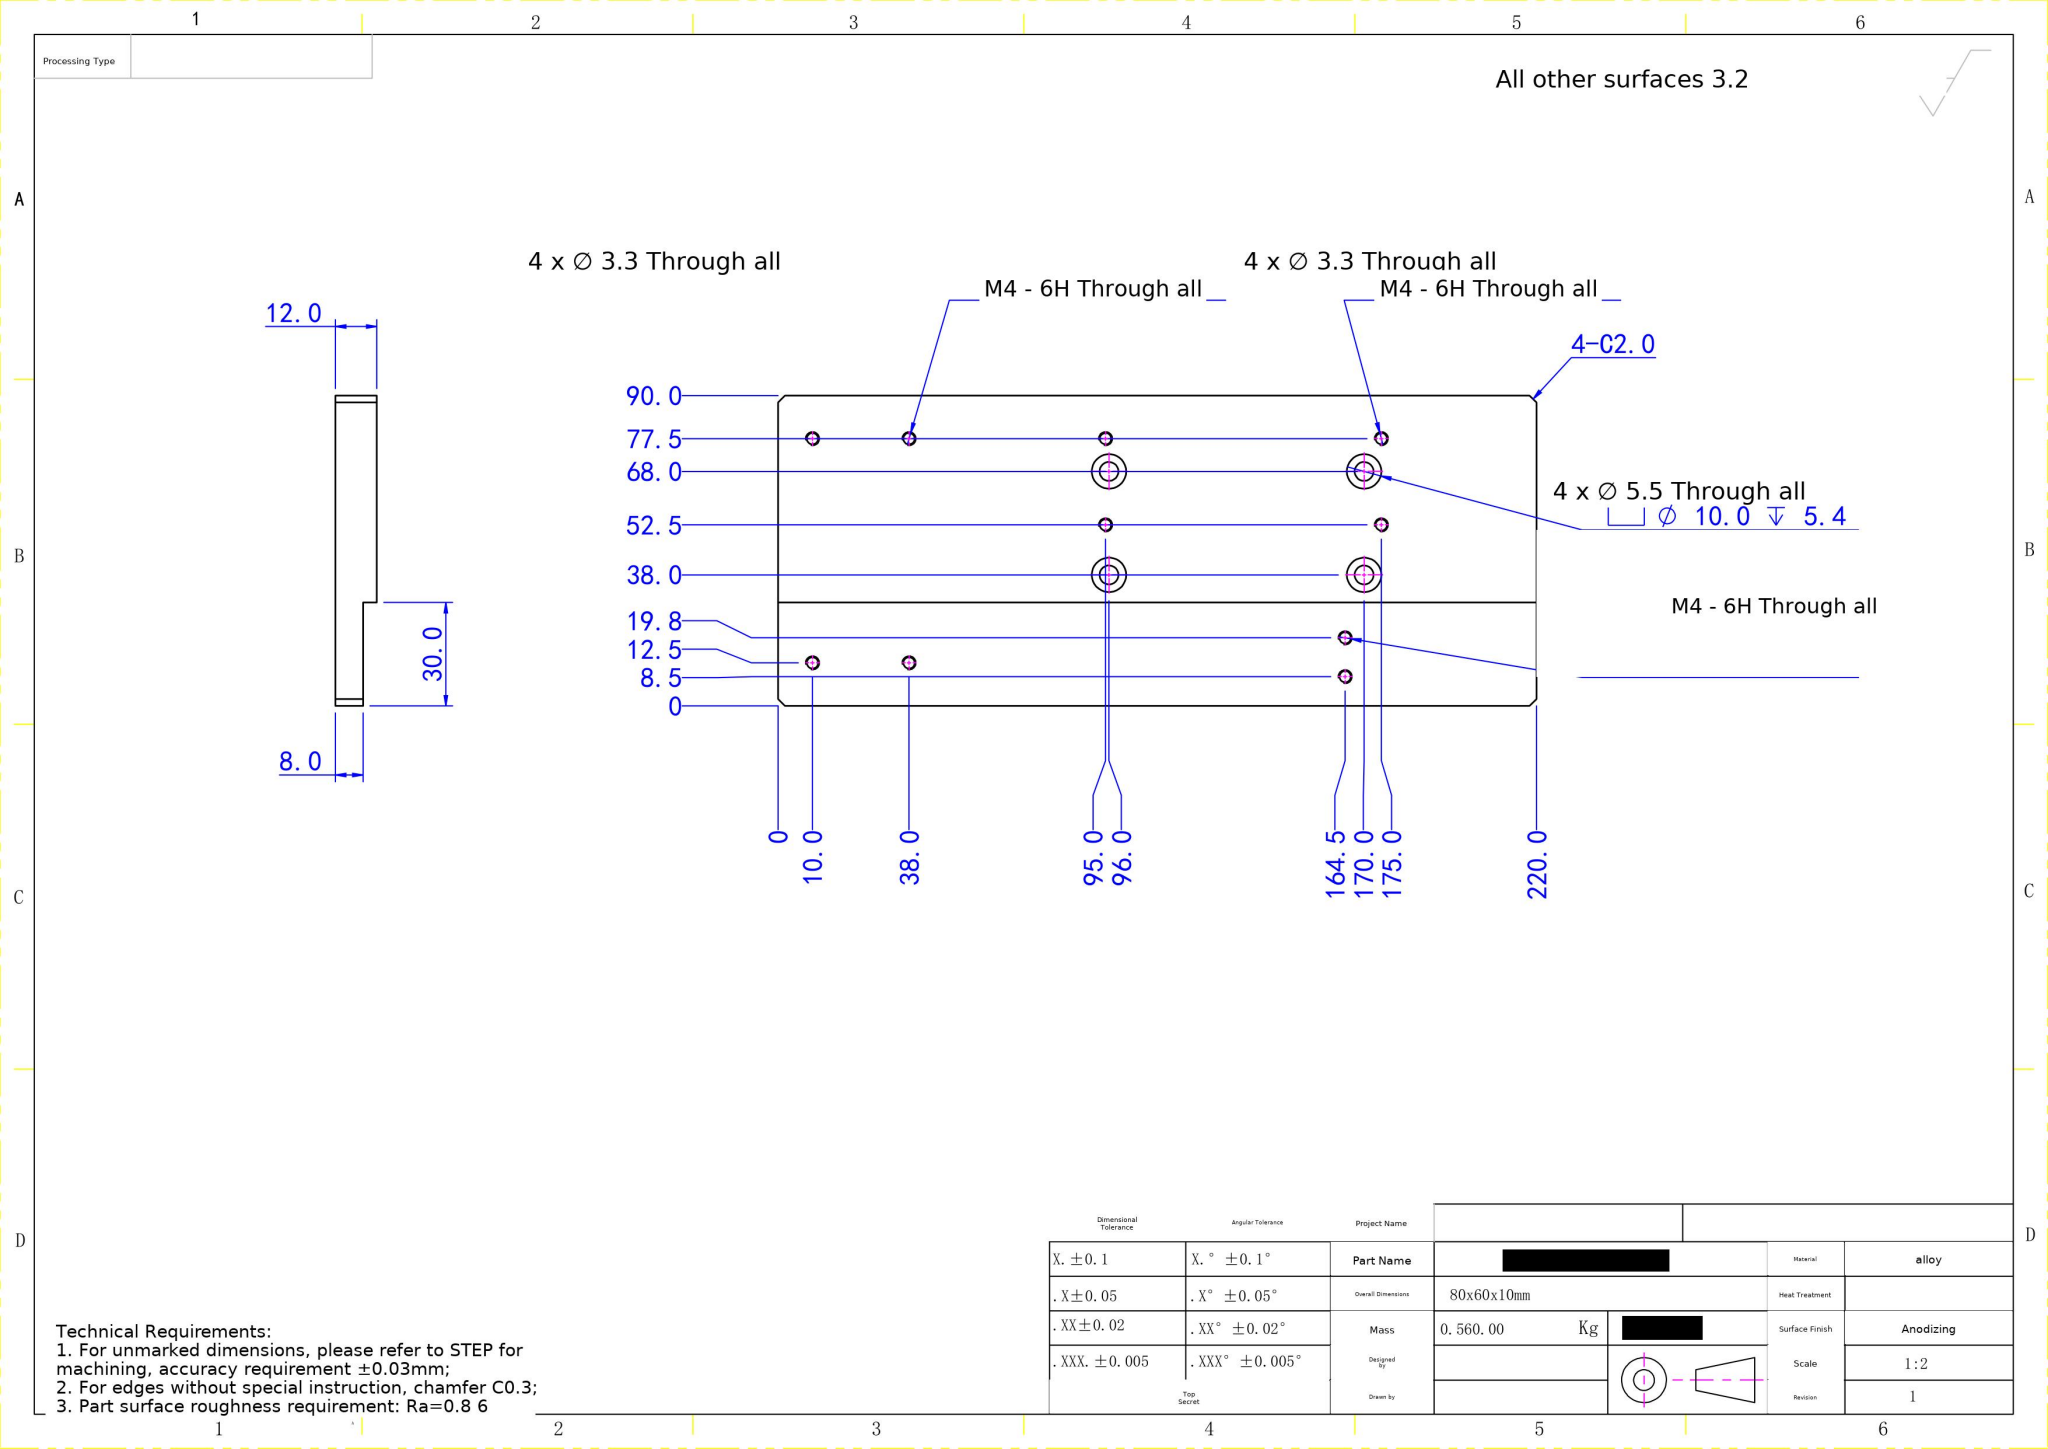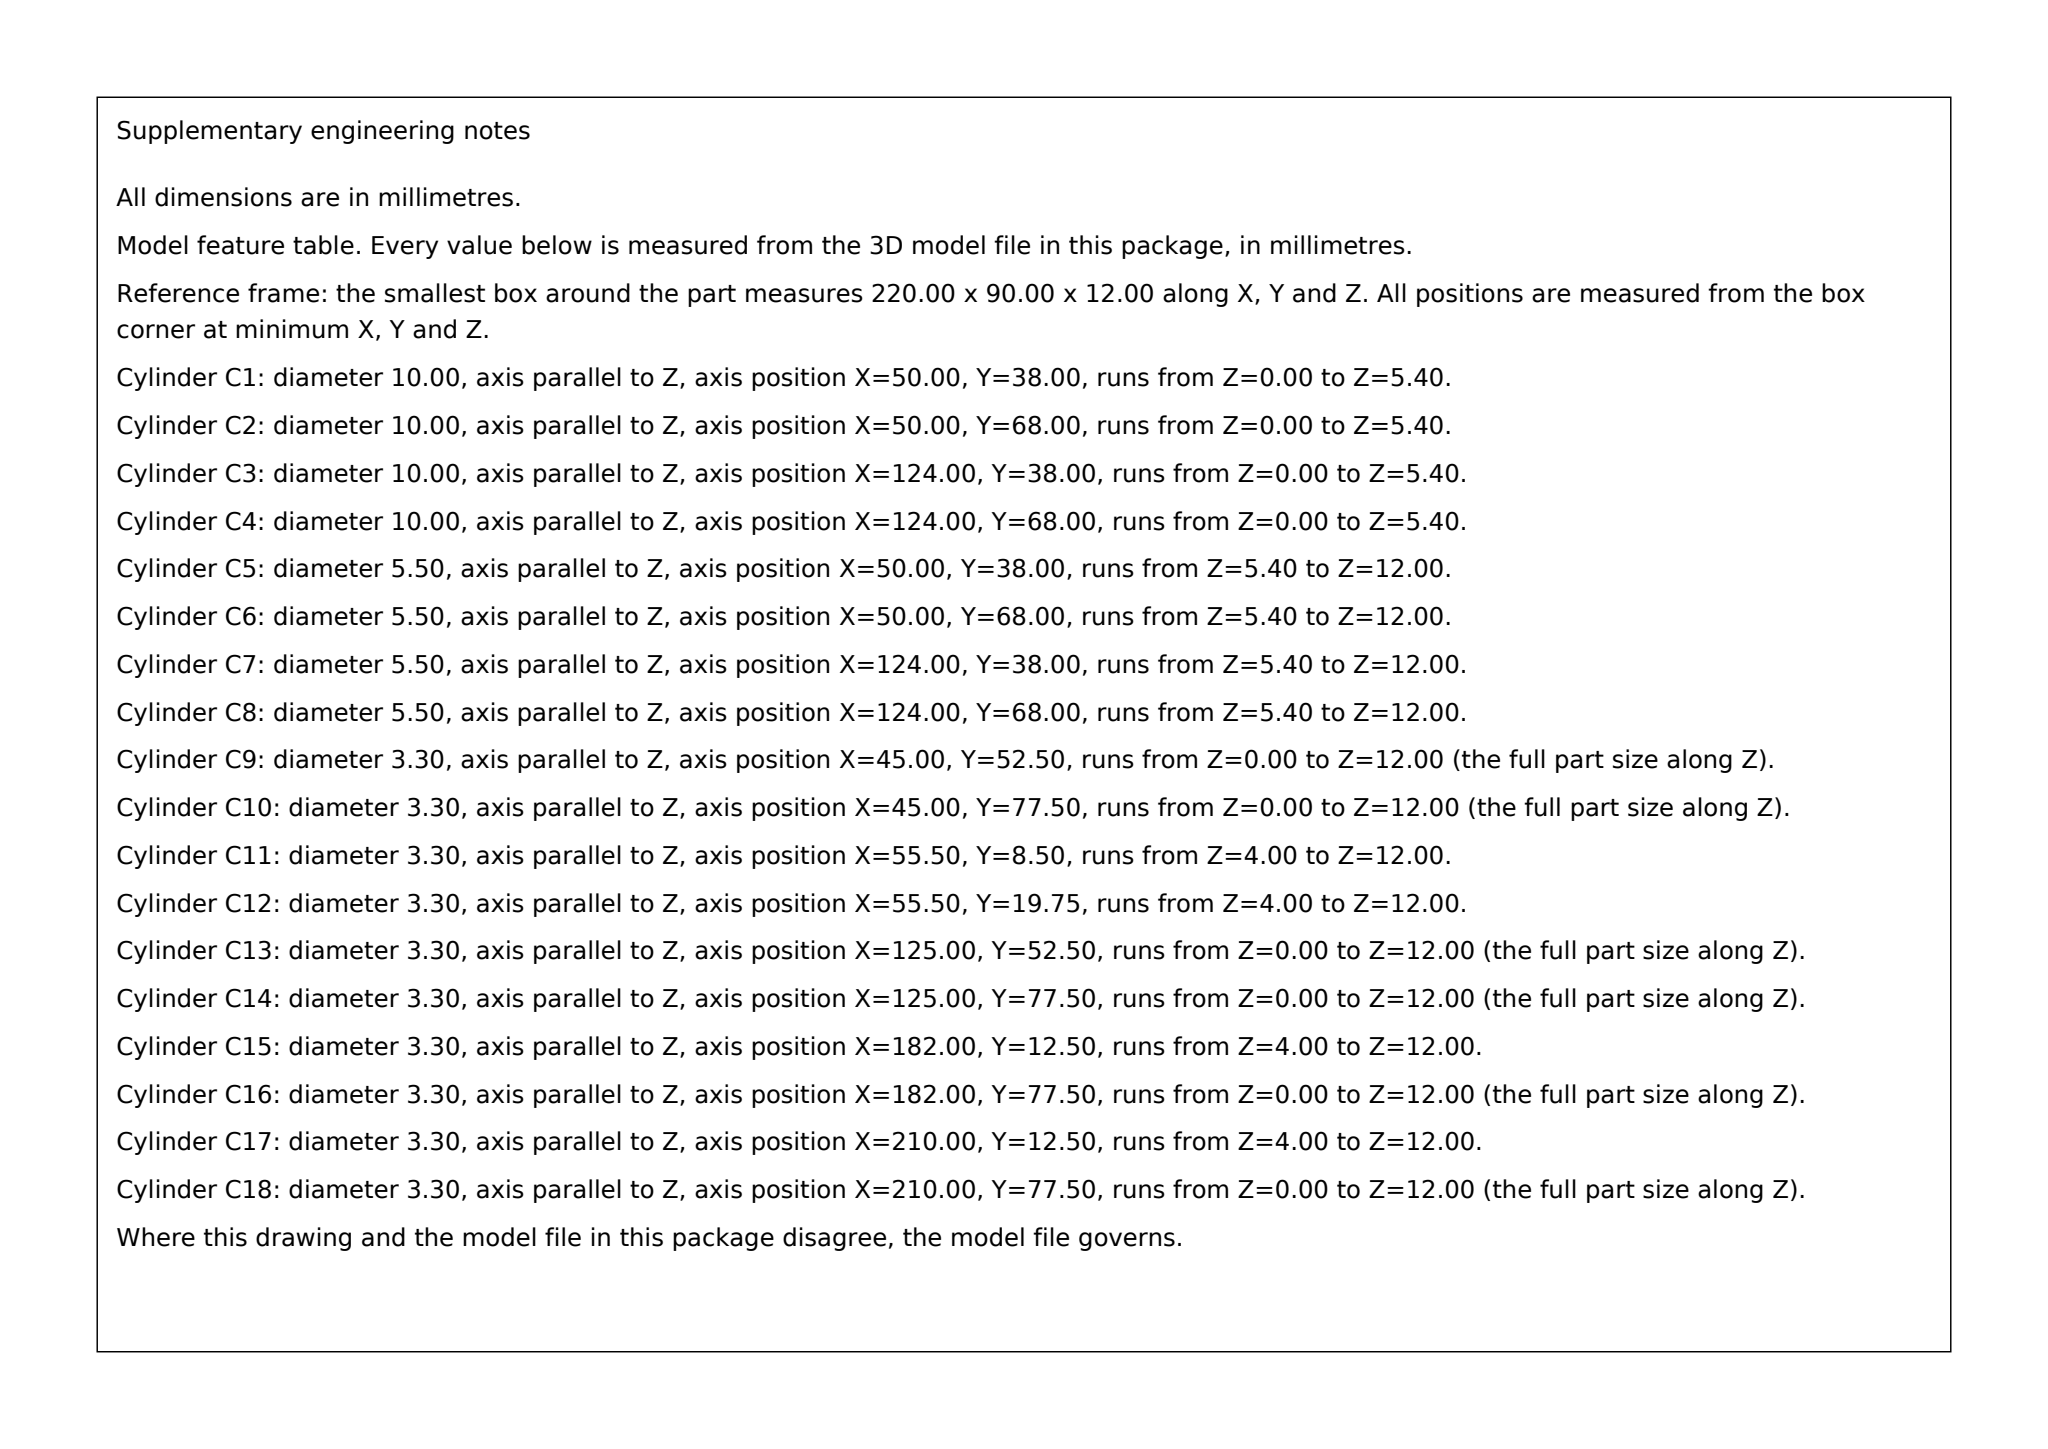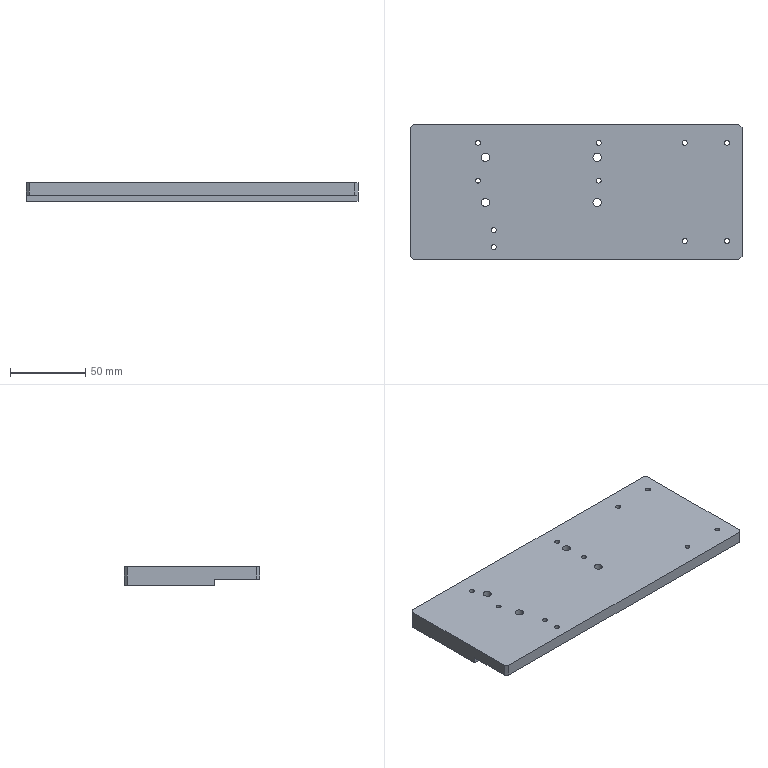Part | SolidWorks | mm | material alloy | 1 solid | 52 faces | box 220 x 90 x 12 mm | volume 207907 mm3 | cylinder 36 | plane 16 | commonest cylinder face diameters 3.3 x20 10 x8 5.5 x8
build123d program:
from build123d import *

# Parameters (mm, degrees)
SKETCH1_W                                       = 220
SKETCH1_H                                       = 90
BOSS_EXTRUDE1_DEPTH                             = 12
M4_TAPPED_HOLE1_D                               = 3.3
M4_TAPPED_HOLE2_D                               = 3.3
M4_TAPPED_HOLE3_D                               = 3.3
M5_HEX_SOCKET_HEAD_CAP_SCREW_CBORE1_D           = 5.5
M5_HEX_SOCKET_HEAD_CAP_SCREW_CBORE1_CBORE_D     = 10
M5_HEX_SOCKET_HEAD_CAP_SCREW_CBORE1_CBORE_DEPTH = 5.4
SKETCH10_W                                      = 220
SKETCH10_H                                      = 30
CUT_EXTRUDE1_DEPTH                              = 4
CHAMFER1_SIZE                                   = 2


with BuildPart() as part:
    # Sketch1 → Boss-Extrude1 (new body)
    with BuildSketch(Plane.XY):
        with Locations((110, 45)):
            Rectangle(SKETCH1_W, SKETCH1_H)
    extrude(amount=BOSS_EXTRUDE1_DEPTH)

    # M4 Tapped Hole1 (through all)
    with Locations(Plane.XY.offset(12)):
        with Locations((182, 77.5), (210, 77.5), (182, 12.5), (210, 12.5)):
            Hole(M4_TAPPED_HOLE1_D / 2)

    # M4 Tapped Hole2 (through all)
    with Locations(Plane(origin=(0, 0, 0), x_dir=(-1, 0, 0), z_dir=(0, 0, -1))):
        with Locations((-55.5, 19.75), (-55.5, 8.5)):
            Hole(M4_TAPPED_HOLE2_D / 2)

    # M4 Tapped Hole3 (through all)
    with Locations(Plane(origin=(0, 0, 0), x_dir=(-1, 0, 0), z_dir=(0, 0, -1))):
        with Locations((-125, 77.5), (-125, 52.5), (-45, 77.5), (-45, 52.5)):
            Hole(M4_TAPPED_HOLE3_D / 2)

    # M5 Hex Socket Head Cap Screw CBORE1 (through all)
    with Locations(Plane(origin=(0, 0, 0), x_dir=(-1, 0, 0), z_dir=(0, 0, -1))):
        with Locations((-124, 38), (-124, 68), (-50, 38), (-50, 68)):
            CounterBoreHole(M5_HEX_SOCKET_HEAD_CAP_SCREW_CBORE1_D / 2, M5_HEX_SOCKET_HEAD_CAP_SCREW_CBORE1_CBORE_D / 2, M5_HEX_SOCKET_HEAD_CAP_SCREW_CBORE1_CBORE_DEPTH)

    # Sketch10 → Cut-Extrude1 (cut)
    with BuildSketch(Plane(origin=(0, 0, 0), x_dir=(-1, 0, 0), z_dir=(0, 0, -1))):
        with Locations((-110, 15)):
            Rectangle(SKETCH10_W, SKETCH10_H)
    extrude(amount=-CUT_EXTRUDE1_DEPTH, mode=Mode.SUBTRACT)

    # Chamfer1
    chamfer1_edges = [part.edges().sort_by_distance(p)[0] for p in [
        (0, 90, 6),
        (220, 90, 6),
        (220, 0, 8),
        (0, 0, 8),
    ]]
    chamfer(chamfer1_edges, length=CHAMFER1_SIZE)


solid = part.part